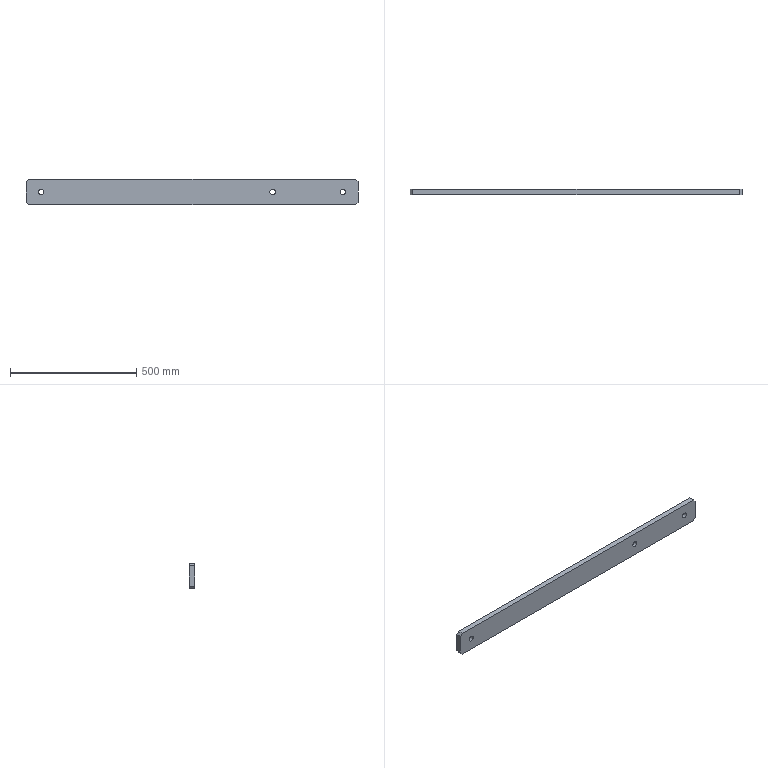Component | SolidWorks | ConnectingRod-1 | 1 solid | 16 faces | box 1315 x 20 x 100 mm | volume 2603192 mm3 | plane 10 | cylinder 6 | commonest cylinder face diameters 22 x6
build123d program:
from build123d import *

# Parameters (mm, degrees)
SKETCH1_W           = 1315
SKETCH1_H           = 100
SKETCH1_R           = 11
BOSS_EXTRUDE1_DEPTH = 20
CHAMFER1_SIZE       = 10


with BuildPart() as part:
    # Sketch1 → Boss-Extrude1 (new body)
    with BuildSketch(Plane.XY):
        Rectangle(SKETCH1_W, SKETCH1_H)
        with Locations((-597.5, 0)):
            Circle(SKETCH1_R, mode=Mode.SUBTRACT)
        with Locations((597.5, 0)):
            Circle(SKETCH1_R, mode=Mode.SUBTRACT)
        with Locations((319.5, 0)):
            Circle(SKETCH1_R, mode=Mode.SUBTRACT)
    extrude(amount=BOSS_EXTRUDE1_DEPTH)

    # Chamfer1
    chamfer1_edges = [part.edges().sort_by_distance(p)[0] for p in [
        (657.5, -50, 10),
        (-657.5, -50, 10),
        (-657.5, 50, 10),
        (657.5, 50, 10),
    ]]
    chamfer(chamfer1_edges, length=CHAMFER1_SIZE)


solid = part.part

# Placed as in the assembly
solid = solid.moved(Location((-319.5, -398, -160), (90, 0, 0)))
STEP:
#1=COLOUR_RGB('',0.7922,0.8196,0.9333);
#2=FILL_AREA_STYLE_COLOUR('',#1);
#3=FILL_AREA_STYLE('',(#2));
#4=SURFACE_STYLE_FILL_AREA(#3);
#5=SURFACE_SIDE_STYLE('',(#4));
#6=SURFACE_STYLE_USAGE(.BOTH.,#5);
#7=PRESENTATION_STYLE_ASSIGNMENT((#6));
#8=CARTESIAN_POINT('',(-0.4331,-15.669,-6.299));
#9=VERTEX_POINT('',#8);
#10=CARTESIAN_POINT('',(0.4331,-15.669,-6.299));
#11=VERTEX_POINT('',#10);
#12=CARTESIAN_POINT('',(-0.,-15.669,-6.299));
#13=DIRECTION('',(0.,1.,0.));
#14=DIRECTION('',(1.,0.,0.));
#15=AXIS2_PLACEMENT_3D('',#12,#13,#14);
#16=CIRCLE('',#15,0.4331);
#17=EDGE_CURVE('',#9,#11,#16,.T.);
#18=ORIENTED_EDGE('',*,*,#17,.T.);
#19=CARTESIAN_POINT('',(0.4331,-16.457,-6.299));
#20=VERTEX_POINT('',#19);
#21=CARTESIAN_POINT('',(0.4331,-15.669,-6.299));
#22=DIRECTION('',(-0.,-1.,-0.));
#23=VECTOR('',#22,39.37);
#24=LINE('',#21,#23);
#25=EDGE_CURVE('',#11,#20,#24,.T.);
#26=ORIENTED_EDGE('',*,*,#25,.T.);
#27=CARTESIAN_POINT('',(-0.4331,-16.457,-6.299));
#28=VERTEX_POINT('',#27);
#29=CARTESIAN_POINT('',(-0.,-16.457,-6.299));
#30=DIRECTION('',(0.,1.,0.));
#31=DIRECTION('',(1.,0.,0.));
#32=AXIS2_PLACEMENT_3D('',#29,#30,#31);
#33=CIRCLE('',#32,0.4331);
#34=EDGE_CURVE('',#28,#20,#33,.T.);
#35=ORIENTED_EDGE('',*,*,#34,.F.);
#36=CARTESIAN_POINT('',(-0.4331,-15.669,-6.299));
#37=DIRECTION('',(-0.,-1.,-0.));
#38=VECTOR('',#37,39.37);
#39=LINE('',#36,#38);
#40=EDGE_CURVE('',#9,#28,#39,.T.);
#41=ORIENTED_EDGE('',*,*,#40,.F.);
#42=EDGE_LOOP('',(#18,#26,#35,#41));
#43=FACE_OUTER_BOUND('',#42,.T.);
#44=CARTESIAN_POINT('',(-0.,-15.669,-6.299));
#45=DIRECTION('',(-0.,-1.,-0.));
#46=DIRECTION('',(-1.,0.,0.));
#47=AXIS2_PLACEMENT_3D('',#44,#45,#46);
#48=CYLINDRICAL_SURFACE('',#47,0.4331);
#49=ADVANCED_FACE('',(#43),#48,.F.);
#50=CARTESIAN_POINT('',(10.512,-15.669,-6.299));
#51=VERTEX_POINT('',#50);
#52=CARTESIAN_POINT('',(11.378,-15.669,-6.299));
#53=VERTEX_POINT('',#52);
#54=CARTESIAN_POINT('',(10.945,-15.669,-6.299));
#55=DIRECTION('',(0.,1.,0.));
#56=DIRECTION('',(1.,0.,0.));
#57=AXIS2_PLACEMENT_3D('',#54,#55,#56);
#58=CIRCLE('',#57,0.4331);
#59=EDGE_CURVE('',#51,#53,#58,.T.);
#60=ORIENTED_EDGE('',*,*,#59,.T.);
#61=CARTESIAN_POINT('',(11.378,-16.457,-6.299));
#62=VERTEX_POINT('',#61);
#63=CARTESIAN_POINT('',(11.378,-15.669,-6.299));
#64=DIRECTION('',(-0.,-1.,-0.));
#65=VECTOR('',#64,39.37);
#66=LINE('',#63,#65);
#67=EDGE_CURVE('',#53,#62,#66,.T.);
#68=ORIENTED_EDGE('',*,*,#67,.T.);
#69=CARTESIAN_POINT('',(10.512,-16.457,-6.299));
#70=VERTEX_POINT('',#69);
#71=CARTESIAN_POINT('',(10.945,-16.457,-6.299));
#72=DIRECTION('',(0.,1.,0.));
#73=DIRECTION('',(1.,0.,0.));
#74=AXIS2_PLACEMENT_3D('',#71,#72,#73);
#75=CIRCLE('',#74,0.4331);
#76=EDGE_CURVE('',#70,#62,#75,.T.);
#77=ORIENTED_EDGE('',*,*,#76,.F.);
#78=CARTESIAN_POINT('',(10.512,-15.669,-6.299));
#79=DIRECTION('',(-0.,-1.,-0.));
#80=VECTOR('',#79,39.37);
#81=LINE('',#78,#80);
#82=EDGE_CURVE('',#51,#70,#81,.T.);
#83=ORIENTED_EDGE('',*,*,#82,.F.);
#84=EDGE_LOOP('',(#60,#68,#77,#83));
#85=FACE_OUTER_BOUND('',#84,.T.);
#86=CARTESIAN_POINT('',(10.945,-15.669,-6.299));
#87=DIRECTION('',(-0.,-1.,-0.));
#88=DIRECTION('',(-1.,0.,0.));
#89=AXIS2_PLACEMENT_3D('',#86,#87,#88);
#90=CYLINDRICAL_SURFACE('',#89,0.4331);
#91=ADVANCED_FACE('',(#85),#90,.F.);
#92=CARTESIAN_POINT('',(-36.535,-15.669,-6.299));
#93=VERTEX_POINT('',#92);
#94=CARTESIAN_POINT('',(-35.669,-15.669,-6.299));
#95=VERTEX_POINT('',#94);
#96=CARTESIAN_POINT('',(-36.102,-15.669,-6.299));
#97=DIRECTION('',(0.,1.,0.));
#98=DIRECTION('',(1.,0.,0.));
#99=AXIS2_PLACEMENT_3D('',#96,#97,#98);
#100=CIRCLE('',#99,0.4331);
#101=EDGE_CURVE('',#93,#95,#100,.T.);
#102=ORIENTED_EDGE('',*,*,#101,.T.);
#103=CARTESIAN_POINT('',(-35.669,-16.457,-6.299));
#104=VERTEX_POINT('',#103);
#105=CARTESIAN_POINT('',(-35.669,-15.669,-6.299));
#106=DIRECTION('',(-0.,-1.,-0.));
#107=VECTOR('',#106,39.37);
#108=LINE('',#105,#107);
#109=EDGE_CURVE('',#95,#104,#108,.T.);
#110=ORIENTED_EDGE('',*,*,#109,.T.);
#111=CARTESIAN_POINT('',(-36.535,-16.457,-6.299));
#112=VERTEX_POINT('',#111);
#113=CARTESIAN_POINT('',(-36.102,-16.457,-6.299));
#114=DIRECTION('',(0.,1.,0.));
#115=DIRECTION('',(1.,0.,0.));
#116=AXIS2_PLACEMENT_3D('',#113,#114,#115);
#117=CIRCLE('',#116,0.4331);
#118=EDGE_CURVE('',#112,#104,#117,.T.);
#119=ORIENTED_EDGE('',*,*,#118,.F.);
#120=CARTESIAN_POINT('',(-36.535,-15.669,-6.299));
#121=DIRECTION('',(-0.,-1.,-0.));
#122=VECTOR('',#121,39.37);
#123=LINE('',#120,#122);
#124=EDGE_CURVE('',#93,#112,#123,.T.);
#125=ORIENTED_EDGE('',*,*,#124,.F.);
#126=EDGE_LOOP('',(#102,#110,#119,#125));
#127=FACE_OUTER_BOUND('',#126,.T.);
#128=CARTESIAN_POINT('',(-36.102,-15.669,-6.299));
#129=DIRECTION('',(-0.,-1.,-0.));
#130=DIRECTION('',(-1.,0.,0.));
#131=AXIS2_PLACEMENT_3D('',#128,#129,#130);
#132=CYLINDRICAL_SURFACE('',#131,0.4331);
#133=ADVANCED_FACE('',(#127),#132,.F.);
#134=ORIENTED_EDGE('',*,*,#59,.F.);
#135=CARTESIAN_POINT('',(10.945,-15.669,-6.299));
#136=DIRECTION('',(0.,1.,0.));
#137=DIRECTION('',(1.,0.,0.));
#138=AXIS2_PLACEMENT_3D('',#135,#136,#137);
#139=CIRCLE('',#138,0.4331);
#140=EDGE_CURVE('',#53,#51,#139,.T.);
#141=ORIENTED_EDGE('',*,*,#140,.F.);
#142=EDGE_LOOP('',(#134,#141));
#143=FACE_BOUND('',#142,.T.);
#144=CARTESIAN_POINT('',(-38.071,-15.669,-4.331));
#145=VERTEX_POINT('',#144);
#146=CARTESIAN_POINT('',(12.913,-15.669,-4.331));
#147=VERTEX_POINT('',#146);
#148=CARTESIAN_POINT('',(-38.465,-15.669,-4.331));
#149=DIRECTION('',(1.,-0.,-0.));
#150=VECTOR('',#149,39.37);
#151=LINE('',#148,#150);
#152=EDGE_CURVE('',#145,#147,#151,.T.);
#153=ORIENTED_EDGE('',*,*,#152,.T.);
#154=CARTESIAN_POINT('',(13.307,-15.669,-4.724));
#155=VERTEX_POINT('',#154);
#156=CARTESIAN_POINT('',(13.307,-15.669,-4.724));
#157=DIRECTION('',(0.7071,-0.,-0.7071));
#158=VECTOR('',#157,39.37);
#159=LINE('',#156,#158);
#160=EDGE_CURVE('',#147,#155,#159,.T.);
#161=ORIENTED_EDGE('',*,*,#160,.T.);
#162=CARTESIAN_POINT('',(13.307,-15.669,-7.874));
#163=VERTEX_POINT('',#162);
#164=CARTESIAN_POINT('',(13.307,-15.669,-4.331));
#165=DIRECTION('',(0.,0.,-1.));
#166=VECTOR('',#165,39.37);
#167=LINE('',#164,#166);
#168=EDGE_CURVE('',#155,#163,#167,.T.);
#169=ORIENTED_EDGE('',*,*,#168,.T.);
#170=CARTESIAN_POINT('',(12.913,-15.669,-8.268));
#171=VERTEX_POINT('',#170);
#172=CARTESIAN_POINT('',(12.913,-15.669,-8.268));
#173=DIRECTION('',(-0.7071,0.,-0.7071));
#174=VECTOR('',#173,39.37);
#175=LINE('',#172,#174);
#176=EDGE_CURVE('',#163,#171,#175,.T.);
#177=ORIENTED_EDGE('',*,*,#176,.T.);
#178=CARTESIAN_POINT('',(-38.071,-15.669,-8.268));
#179=VERTEX_POINT('',#178);
#180=CARTESIAN_POINT('',(-38.465,-15.669,-8.268));
#181=DIRECTION('',(-1.,0.,0.));
#182=VECTOR('',#181,39.37);
#183=LINE('',#180,#182);
#184=EDGE_CURVE('',#171,#179,#183,.T.);
#185=ORIENTED_EDGE('',*,*,#184,.T.);
#186=CARTESIAN_POINT('',(-38.465,-15.669,-7.874));
#187=VERTEX_POINT('',#186);
#188=CARTESIAN_POINT('',(-38.465,-15.669,-7.874));
#189=DIRECTION('',(-0.7071,0.,0.7071));
#190=VECTOR('',#189,39.37);
#191=LINE('',#188,#190);
#192=EDGE_CURVE('',#179,#187,#191,.T.);
#193=ORIENTED_EDGE('',*,*,#192,.T.);
#194=CARTESIAN_POINT('',(-38.465,-15.669,-4.724));
#195=VERTEX_POINT('',#194);
#196=CARTESIAN_POINT('',(-38.465,-15.669,-4.331));
#197=DIRECTION('',(0.,-0.,1.));
#198=VECTOR('',#197,39.37);
#199=LINE('',#196,#198);
#200=EDGE_CURVE('',#187,#195,#199,.T.);
#201=ORIENTED_EDGE('',*,*,#200,.T.);
#202=CARTESIAN_POINT('',(-38.071,-15.669,-4.331));
#203=DIRECTION('',(0.7071,-0.,0.7071));
#204=VECTOR('',#203,39.37);
#205=LINE('',#202,#204);
#206=EDGE_CURVE('',#195,#145,#205,.T.);
#207=ORIENTED_EDGE('',*,*,#206,.T.);
#208=EDGE_LOOP('',(#153,#161,#169,#177,#185,#193,#201,#207));
#209=FACE_OUTER_BOUND('',#208,.T.);
#210=ORIENTED_EDGE('',*,*,#101,.F.);
#211=CARTESIAN_POINT('',(-36.102,-15.669,-6.299));
#212=DIRECTION('',(0.,1.,0.));
#213=DIRECTION('',(1.,0.,0.));
#214=AXIS2_PLACEMENT_3D('',#211,#212,#213);
#215=CIRCLE('',#214,0.4331);
#216=EDGE_CURVE('',#95,#93,#215,.T.);
#217=ORIENTED_EDGE('',*,*,#216,.F.);
#218=EDGE_LOOP('',(#210,#217));
#219=FACE_BOUND('',#218,.T.);
#220=ORIENTED_EDGE('',*,*,#17,.F.);
#221=CARTESIAN_POINT('',(-0.,-15.669,-6.299));
#222=DIRECTION('',(0.,1.,0.));
#223=DIRECTION('',(1.,0.,0.));
#224=AXIS2_PLACEMENT_3D('',#221,#222,#223);
#225=CIRCLE('',#224,0.4331);
#226=EDGE_CURVE('',#11,#9,#225,.T.);
#227=ORIENTED_EDGE('',*,*,#226,.F.);
#228=EDGE_LOOP('',(#220,#227));
#229=FACE_BOUND('',#228,.T.);
#230=CARTESIAN_POINT('',(-12.579,-15.669,-6.299));
#231=DIRECTION('',(-0.,-1.,-0.));
#232=DIRECTION('',(-1.,0.,0.));
#233=AXIS2_PLACEMENT_3D('',#230,#231,#232);
#234=PLANE('',#233);
#235=ADVANCED_FACE('',(#143,#209,#219,#229),#234,.F.);
#236=ORIENTED_EDGE('',*,*,#76,.T.);
#237=CARTESIAN_POINT('',(10.945,-16.457,-6.299));
#238=DIRECTION('',(0.,1.,0.));
#239=DIRECTION('',(1.,0.,0.));
#240=AXIS2_PLACEMENT_3D('',#237,#238,#239);
#241=CIRCLE('',#240,0.4331);
#242=EDGE_CURVE('',#62,#70,#241,.T.);
#243=ORIENTED_EDGE('',*,*,#242,.T.);
#244=EDGE_LOOP('',(#236,#243));
#245=FACE_BOUND('',#244,.T.);
#246=CARTESIAN_POINT('',(13.307,-16.457,-4.724));
#247=VERTEX_POINT('',#246);
#248=CARTESIAN_POINT('',(13.307,-16.457,-7.874));
#249=VERTEX_POINT('',#248);
#250=CARTESIAN_POINT('',(13.307,-16.457,-4.331));
#251=DIRECTION('',(0.,0.,-1.));
#252=VECTOR('',#251,39.37);
#253=LINE('',#250,#252);
#254=EDGE_CURVE('',#247,#249,#253,.T.);
#255=ORIENTED_EDGE('',*,*,#254,.F.);
#256=CARTESIAN_POINT('',(12.913,-16.457,-4.331));
#257=VERTEX_POINT('',#256);
#258=CARTESIAN_POINT('',(1.152,-16.457,7.431));
#259=DIRECTION('',(-0.7071,0.,0.7071));
#260=VECTOR('',#259,39.37);
#261=LINE('',#258,#260);
#262=EDGE_CURVE('',#247,#257,#261,.T.);
#263=ORIENTED_EDGE('',*,*,#262,.T.);
#264=CARTESIAN_POINT('',(-38.071,-16.457,-4.331));
#265=VERTEX_POINT('',#264);
#266=CARTESIAN_POINT('',(-38.465,-16.457,-4.331));
#267=DIRECTION('',(1.,-0.,-0.));
#268=VECTOR('',#267,39.37);
#269=LINE('',#266,#268);
#270=EDGE_CURVE('',#265,#257,#269,.T.);
#271=ORIENTED_EDGE('',*,*,#270,.F.);
#272=CARTESIAN_POINT('',(-38.465,-16.457,-4.724));
#273=VERTEX_POINT('',#272);
#274=CARTESIAN_POINT('',(-26.309,-16.457,7.431));
#275=DIRECTION('',(-0.7071,0.,-0.7071));
#276=VECTOR('',#275,39.37);
#277=LINE('',#274,#276);
#278=EDGE_CURVE('',#265,#273,#277,.T.);
#279=ORIENTED_EDGE('',*,*,#278,.T.);
#280=CARTESIAN_POINT('',(-38.465,-16.457,-7.874));
#281=VERTEX_POINT('',#280);
#282=CARTESIAN_POINT('',(-38.465,-16.457,-4.331));
#283=DIRECTION('',(0.,-0.,1.));
#284=VECTOR('',#283,39.37);
#285=LINE('',#282,#284);
#286=EDGE_CURVE('',#281,#273,#285,.T.);
#287=ORIENTED_EDGE('',*,*,#286,.F.);
#288=CARTESIAN_POINT('',(-38.071,-16.457,-8.268));
#289=VERTEX_POINT('',#288);
#290=CARTESIAN_POINT('',(-26.309,-16.457,-20.03));
#291=DIRECTION('',(0.7071,-0.,-0.7071));
#292=VECTOR('',#291,39.37);
#293=LINE('',#290,#292);
#294=EDGE_CURVE('',#281,#289,#293,.T.);
#295=ORIENTED_EDGE('',*,*,#294,.T.);
#296=CARTESIAN_POINT('',(12.913,-16.457,-8.268));
#297=VERTEX_POINT('',#296);
#298=CARTESIAN_POINT('',(-38.465,-16.457,-8.268));
#299=DIRECTION('',(-1.,0.,0.));
#300=VECTOR('',#299,39.37);
#301=LINE('',#298,#300);
#302=EDGE_CURVE('',#297,#289,#301,.T.);
#303=ORIENTED_EDGE('',*,*,#302,.F.);
#304=CARTESIAN_POINT('',(1.152,-16.457,-20.03));
#305=DIRECTION('',(0.7071,-0.,0.7071));
#306=VECTOR('',#305,39.37);
#307=LINE('',#304,#306);
#308=EDGE_CURVE('',#297,#249,#307,.T.);
#309=ORIENTED_EDGE('',*,*,#308,.T.);
#310=EDGE_LOOP('',(#255,#263,#271,#279,#287,#295,#303,#309));
#311=FACE_OUTER_BOUND('',#310,.T.);
#312=ORIENTED_EDGE('',*,*,#118,.T.);
#313=CARTESIAN_POINT('',(-36.102,-16.457,-6.299));
#314=DIRECTION('',(0.,1.,0.));
#315=DIRECTION('',(1.,0.,0.));
#316=AXIS2_PLACEMENT_3D('',#313,#314,#315);
#317=CIRCLE('',#316,0.4331);
#318=EDGE_CURVE('',#104,#112,#317,.T.);
#319=ORIENTED_EDGE('',*,*,#318,.T.);
#320=EDGE_LOOP('',(#312,#319));
#321=FACE_BOUND('',#320,.T.);
#322=ORIENTED_EDGE('',*,*,#34,.T.);
#323=CARTESIAN_POINT('',(-0.,-16.457,-6.299));
#324=DIRECTION('',(0.,1.,0.));
#325=DIRECTION('',(1.,0.,0.));
#326=AXIS2_PLACEMENT_3D('',#323,#324,#325);
#327=CIRCLE('',#326,0.4331);
#328=EDGE_CURVE('',#20,#28,#327,.T.);
#329=ORIENTED_EDGE('',*,*,#328,.T.);
#330=EDGE_LOOP('',(#322,#329));
#331=FACE_BOUND('',#330,.T.);
#332=CARTESIAN_POINT('',(-12.579,-16.457,-6.299));
#333=DIRECTION('',(-0.,-1.,-0.));
#334=DIRECTION('',(-1.,0.,0.));
#335=AXIS2_PLACEMENT_3D('',#332,#333,#334);
#336=PLANE('',#335);
#337=ADVANCED_FACE('',(#245,#311,#321,#331),#336,.T.);
#338=ORIENTED_EDGE('',*,*,#168,.F.);
#339=CARTESIAN_POINT('',(13.307,-15.669,-4.724));
#340=DIRECTION('',(-0.,-1.,-0.));
#341=VECTOR('',#340,39.37);
#342=LINE('',#339,#341);
#343=EDGE_CURVE('',#155,#247,#342,.T.);
#344=ORIENTED_EDGE('',*,*,#343,.T.);
#345=ORIENTED_EDGE('',*,*,#254,.T.);
#346=CARTESIAN_POINT('',(13.307,-15.669,-7.874));
#347=DIRECTION('',(0.,1.,0.));
#348=VECTOR('',#347,39.37);
#349=LINE('',#346,#348);
#350=EDGE_CURVE('',#249,#163,#349,.T.);
#351=ORIENTED_EDGE('',*,*,#350,.T.);
#352=EDGE_LOOP('',(#338,#344,#345,#351));
#353=FACE_OUTER_BOUND('',#352,.T.);
#354=CARTESIAN_POINT('',(13.307,-15.669,-4.331));
#355=DIRECTION('',(-1.,0.,0.));
#356=DIRECTION('',(0.,1.,0.));
#357=AXIS2_PLACEMENT_3D('',#354,#355,#356);
#358=PLANE('',#357);
#359=ADVANCED_FACE('',(#353),#358,.F.);
#360=ORIENTED_EDGE('',*,*,#184,.F.);
#361=CARTESIAN_POINT('',(12.913,-15.669,-8.268));
#362=DIRECTION('',(-0.,-1.,-0.));
#363=VECTOR('',#362,39.37);
#364=LINE('',#361,#363);
#365=EDGE_CURVE('',#171,#297,#364,.T.);
#366=ORIENTED_EDGE('',*,*,#365,.T.);
#367=ORIENTED_EDGE('',*,*,#302,.T.);
#368=CARTESIAN_POINT('',(-38.071,-15.669,-8.268));
#369=DIRECTION('',(0.,1.,0.));
#370=VECTOR('',#369,39.37);
#371=LINE('',#368,#370);
#372=EDGE_CURVE('',#289,#179,#371,.T.);
#373=ORIENTED_EDGE('',*,*,#372,.T.);
#374=EDGE_LOOP('',(#360,#366,#367,#373));
#375=FACE_OUTER_BOUND('',#374,.T.);
#376=CARTESIAN_POINT('',(-38.465,-15.669,-8.268));
#377=DIRECTION('',(0.,-0.,1.));
#378=DIRECTION('',(-0.,-1.,-0.));
#379=AXIS2_PLACEMENT_3D('',#376,#377,#378);
#380=PLANE('',#379);
#381=ADVANCED_FACE('',(#375),#380,.F.);
#382=ORIENTED_EDGE('',*,*,#286,.T.);
#383=CARTESIAN_POINT('',(-38.465,-15.669,-4.724));
#384=DIRECTION('',(0.,1.,0.));
#385=VECTOR('',#384,39.37);
#386=LINE('',#383,#385);
#387=EDGE_CURVE('',#273,#195,#386,.T.);
#388=ORIENTED_EDGE('',*,*,#387,.T.);
#389=ORIENTED_EDGE('',*,*,#200,.F.);
#390=CARTESIAN_POINT('',(-38.465,-15.669,-7.874));
#391=DIRECTION('',(-0.,-1.,-0.));
#392=VECTOR('',#391,39.37);
#393=LINE('',#390,#392);
#394=EDGE_CURVE('',#187,#281,#393,.T.);
#395=ORIENTED_EDGE('',*,*,#394,.T.);
#396=EDGE_LOOP('',(#382,#388,#389,#395));
#397=FACE_OUTER_BOUND('',#396,.T.);
#398=CARTESIAN_POINT('',(-38.465,-15.669,-4.331));
#399=DIRECTION('',(1.,-0.,-0.));
#400=DIRECTION('',(-0.,-1.,-0.));
#401=AXIS2_PLACEMENT_3D('',#398,#399,#400);
#402=PLANE('',#401);
#403=ADVANCED_FACE('',(#397),#402,.F.);
#404=ORIENTED_EDGE('',*,*,#270,.T.);
#405=CARTESIAN_POINT('',(12.913,-15.669,-4.331));
#406=DIRECTION('',(0.,1.,0.));
#407=VECTOR('',#406,39.37);
#408=LINE('',#405,#407);
#409=EDGE_CURVE('',#257,#147,#408,.T.);
#410=ORIENTED_EDGE('',*,*,#409,.T.);
#411=ORIENTED_EDGE('',*,*,#152,.F.);
#412=CARTESIAN_POINT('',(-38.071,-15.669,-4.331));
#413=DIRECTION('',(-0.,-1.,-0.));
#414=VECTOR('',#413,39.37);
#415=LINE('',#412,#414);
#416=EDGE_CURVE('',#145,#265,#415,.T.);
#417=ORIENTED_EDGE('',*,*,#416,.T.);
#418=EDGE_LOOP('',(#404,#410,#411,#417));
#419=FACE_OUTER_BOUND('',#418,.T.);
#420=CARTESIAN_POINT('',(-38.465,-15.669,-4.331));
#421=DIRECTION('',(-0.,0.,-1.));
#422=DIRECTION('',(0.,1.,0.));
#423=AXIS2_PLACEMENT_3D('',#420,#421,#422);
#424=PLANE('',#423);
#425=ADVANCED_FACE('',(#419),#424,.F.);
#426=ORIENTED_EDGE('',*,*,#109,.F.);
#427=ORIENTED_EDGE('',*,*,#216,.T.);
#428=ORIENTED_EDGE('',*,*,#124,.T.);
#429=ORIENTED_EDGE('',*,*,#318,.F.);
#430=EDGE_LOOP('',(#426,#427,#428,#429));
#431=FACE_OUTER_BOUND('',#430,.T.);
#432=CARTESIAN_POINT('',(-36.102,-15.669,-6.299));
#433=DIRECTION('',(-0.,-1.,-0.));
#434=DIRECTION('',(-1.,0.,0.));
#435=AXIS2_PLACEMENT_3D('',#432,#433,#434);
#436=CYLINDRICAL_SURFACE('',#435,0.4331);
#437=ADVANCED_FACE('',(#431),#436,.F.);
#438=ORIENTED_EDGE('',*,*,#67,.F.);
#439=ORIENTED_EDGE('',*,*,#140,.T.);
#440=ORIENTED_EDGE('',*,*,#82,.T.);
#441=ORIENTED_EDGE('',*,*,#242,.F.);
#442=EDGE_LOOP('',(#438,#439,#440,#441));
#443=FACE_OUTER_BOUND('',#442,.T.);
#444=CARTESIAN_POINT('',(10.945,-15.669,-6.299));
#445=DIRECTION('',(-0.,-1.,-0.));
#446=DIRECTION('',(-1.,0.,0.));
#447=AXIS2_PLACEMENT_3D('',#444,#445,#446);
#448=CYLINDRICAL_SURFACE('',#447,0.4331);
#449=ADVANCED_FACE('',(#443),#448,.F.);
#450=ORIENTED_EDGE('',*,*,#25,.F.);
#451=ORIENTED_EDGE('',*,*,#226,.T.);
#452=ORIENTED_EDGE('',*,*,#40,.T.);
#453=ORIENTED_EDGE('',*,*,#328,.F.);
#454=EDGE_LOOP('',(#450,#451,#452,#453));
#455=FACE_OUTER_BOUND('',#454,.T.);
#456=CARTESIAN_POINT('',(-0.,-15.669,-6.299));
#457=DIRECTION('',(-0.,-1.,-0.));
#458=DIRECTION('',(-1.,0.,0.));
#459=AXIS2_PLACEMENT_3D('',#456,#457,#458);
#460=CYLINDRICAL_SURFACE('',#459,0.4331);
#461=ADVANCED_FACE('',(#455),#460,.F.);
#462=ORIENTED_EDGE('',*,*,#160,.F.);
#463=ORIENTED_EDGE('',*,*,#409,.F.);
#464=ORIENTED_EDGE('',*,*,#262,.F.);
#465=ORIENTED_EDGE('',*,*,#343,.F.);
#466=EDGE_LOOP('',(#462,#463,#464,#465));
#467=FACE_OUTER_BOUND('',#466,.T.);
#468=CARTESIAN_POINT('',(13.307,-15.669,-4.724));
#469=DIRECTION('',(-0.7071,0.,-0.7071));
#470=DIRECTION('',(-0.,-1.,-0.));
#471=AXIS2_PLACEMENT_3D('',#468,#469,#470);
#472=PLANE('',#471);
#473=ADVANCED_FACE('',(#467),#472,.F.);
#474=ORIENTED_EDGE('',*,*,#176,.F.);
#475=ORIENTED_EDGE('',*,*,#350,.F.);
#476=ORIENTED_EDGE('',*,*,#308,.F.);
#477=ORIENTED_EDGE('',*,*,#365,.F.);
#478=EDGE_LOOP('',(#474,#475,#476,#477));
#479=FACE_OUTER_BOUND('',#478,.T.);
#480=CARTESIAN_POINT('',(12.913,-15.669,-8.268));
#481=DIRECTION('',(-0.7071,0.,0.7071));
#482=DIRECTION('',(-0.,-1.,-0.));
#483=AXIS2_PLACEMENT_3D('',#480,#481,#482);
#484=PLANE('',#483);
#485=ADVANCED_FACE('',(#479),#484,.F.);
#486=ORIENTED_EDGE('',*,*,#206,.F.);
#487=ORIENTED_EDGE('',*,*,#387,.F.);
#488=ORIENTED_EDGE('',*,*,#278,.F.);
#489=ORIENTED_EDGE('',*,*,#416,.F.);
#490=EDGE_LOOP('',(#486,#487,#488,#489));
#491=FACE_OUTER_BOUND('',#490,.T.);
#492=CARTESIAN_POINT('',(-38.071,-15.669,-4.331));
#493=DIRECTION('',(0.7071,-0.,-0.7071));
#494=DIRECTION('',(-0.,-1.,-0.));
#495=AXIS2_PLACEMENT_3D('',#492,#493,#494);
#496=PLANE('',#495);
#497=ADVANCED_FACE('',(#491),#496,.F.);
#498=ORIENTED_EDGE('',*,*,#192,.F.);
#499=ORIENTED_EDGE('',*,*,#372,.F.);
#500=ORIENTED_EDGE('',*,*,#294,.F.);
#501=ORIENTED_EDGE('',*,*,#394,.F.);
#502=EDGE_LOOP('',(#498,#499,#500,#501));
#503=FACE_OUTER_BOUND('',#502,.T.);
#504=CARTESIAN_POINT('',(-38.465,-15.669,-7.874));
#505=DIRECTION('',(0.7071,-0.,0.7071));
#506=DIRECTION('',(-0.,-1.,-0.));
#507=AXIS2_PLACEMENT_3D('',#504,#505,#506);
#508=PLANE('',#507);
#509=ADVANCED_FACE('',(#503),#508,.F.);
#510=CLOSED_SHELL('',(#49,#91,#133,#235,#337,#359,#381,#403,#425,#437,#449,#461,#473,#485,#497,#509));
#511=MANIFOLD_SOLID_BREP('',#510);
#512=STYLED_ITEM('',(#7),#511);
#513=(LENGTH_UNIT()NAMED_UNIT(*)SI_UNIT($,.METRE.));
#514=LENGTH_MEASURE_WITH_UNIT(LENGTH_MEASURE(0.0254),#513);
#515=DIMENSIONAL_EXPONENTS(1.,0.,0.,0.,0.,0.,0.);
#516=(CONVERSION_BASED_UNIT('',#514)LENGTH_UNIT()NAMED_UNIT(#515));
#517=UNCERTAINTY_MEASURE_WITH_UNIT(LENGTH_MEASURE(0.00001),#516,'','');
#518=(NAMED_UNIT(*)PLANE_ANGLE_UNIT()SI_UNIT($,.RADIAN.));
#519=(NAMED_UNIT(*)SI_UNIT($,.STERADIAN.)SOLID_ANGLE_UNIT());
#520=(GEOMETRIC_REPRESENTATION_CONTEXT(3)GLOBAL_UNCERTAINTY_ASSIGNED_CONTEXT((#517))GLOBAL_UNIT_ASSIGNED_CONTEXT((#516,#518,#519))REPRESENTATION_CONTEXT('',''));
#521=MECHANICAL_DESIGN_GEOMETRIC_PRESENTATION_REPRESENTATION('',(#512),#520);
#522=CARTESIAN_POINT('',(0.,0.,0.));
#523=DIRECTION('',(0.,0.,1.));
#524=DIRECTION('',(1.,0.,0.));
#525=AXIS2_PLACEMENT_3D('',#522,#523,#524);
#526=(LENGTH_UNIT()NAMED_UNIT(*)SI_UNIT($,.METRE.));
#527=LENGTH_MEASURE_WITH_UNIT(LENGTH_MEASURE(0.0254),#526);
#528=DIMENSIONAL_EXPONENTS(1.,0.,0.,0.,0.,0.,0.);
#529=(CONVERSION_BASED_UNIT('',#527)LENGTH_UNIT()NAMED_UNIT(#528));
#530=UNCERTAINTY_MEASURE_WITH_UNIT(LENGTH_MEASURE(0.00001),#529,'','');
#531=(NAMED_UNIT(*)PLANE_ANGLE_UNIT()SI_UNIT($,.RADIAN.));
#532=(NAMED_UNIT(*)SI_UNIT($,.STERADIAN.)SOLID_ANGLE_UNIT());
#533=(GEOMETRIC_REPRESENTATION_CONTEXT(3)GLOBAL_UNCERTAINTY_ASSIGNED_CONTEXT((#530))GLOBAL_UNIT_ASSIGNED_CONTEXT((#529,#531,#532))REPRESENTATION_CONTEXT('',''));
#534=ADVANCED_BREP_SHAPE_REPRESENTATION('',(#511,#525),#533);
#535=PRESENTATION_LAYER_ASSIGNMENT('','',(#512));